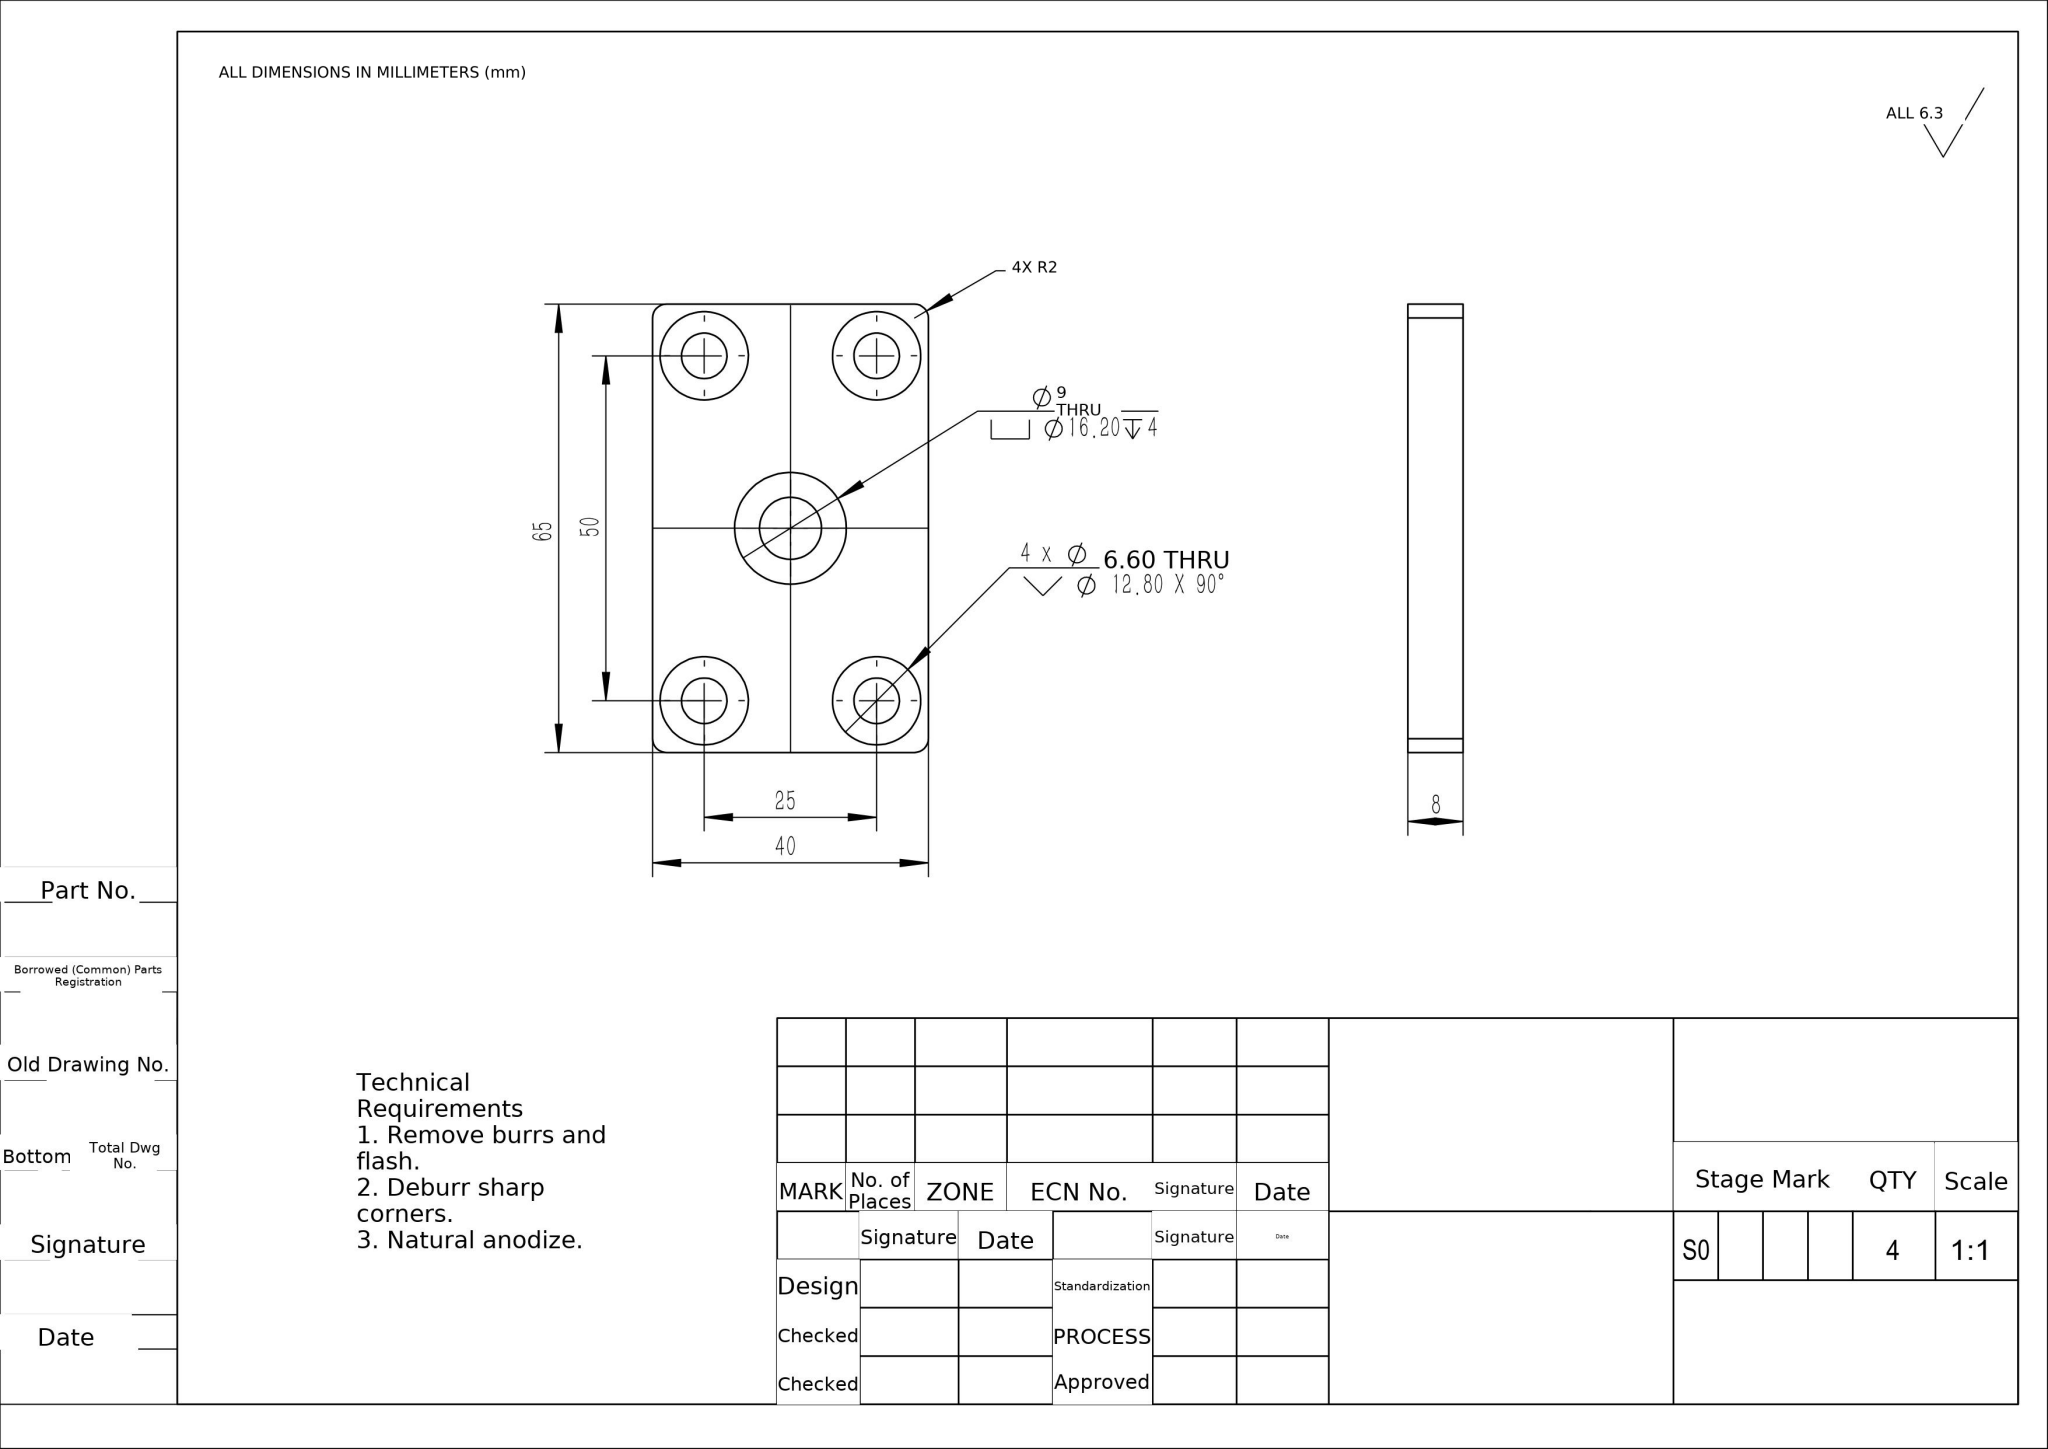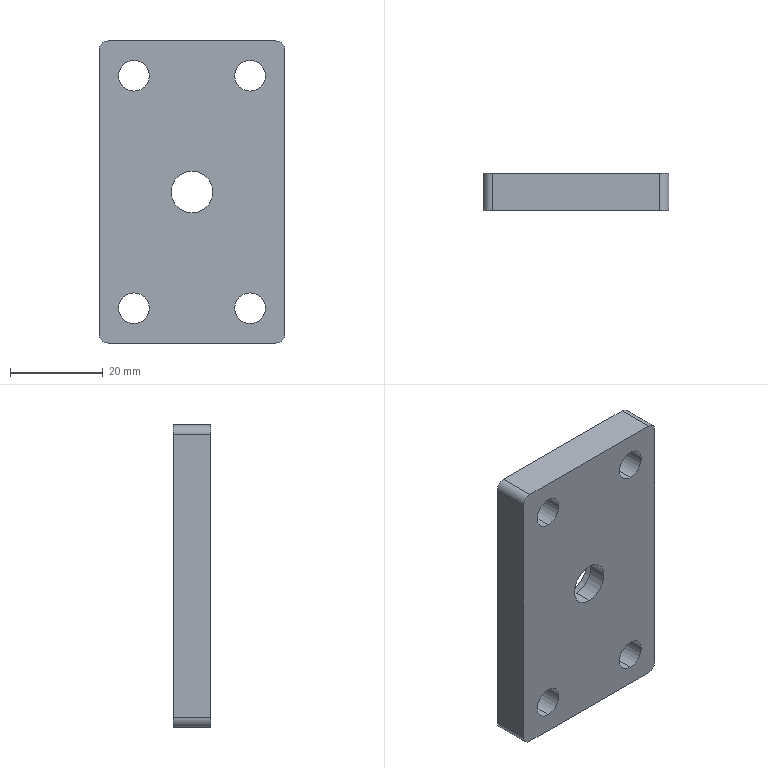Part | NX | mm | 1 solid | 31 faces | box 40 x 8 x 65 mm | volume 18075 mm3 | cylinder 16 | cone 8 | plane 7 | commonest cylinder face diameters 6.6 x8 4 x4 16.2 x2 9 x2